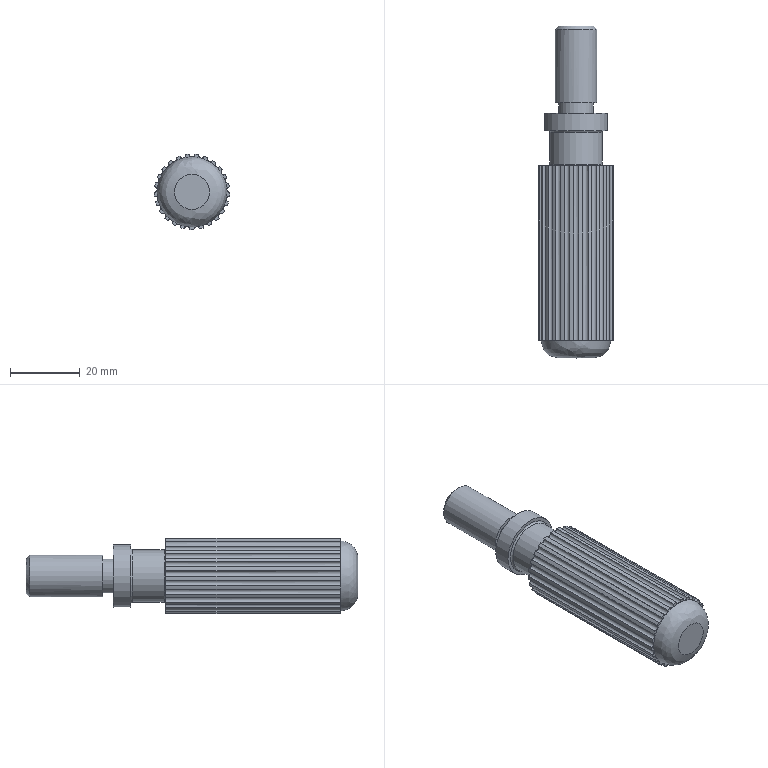Component | NX | LOCATING_PLUG | 1 solid | 89 faces | volume 24107 mm3 | cylinder 54 | plane 31 | torus 2 | spline 1 | cone 1 | commonest cylinder face diameters 21.6 x25 1.6 x25 12 x1 10 x1 18 x1 15 x1